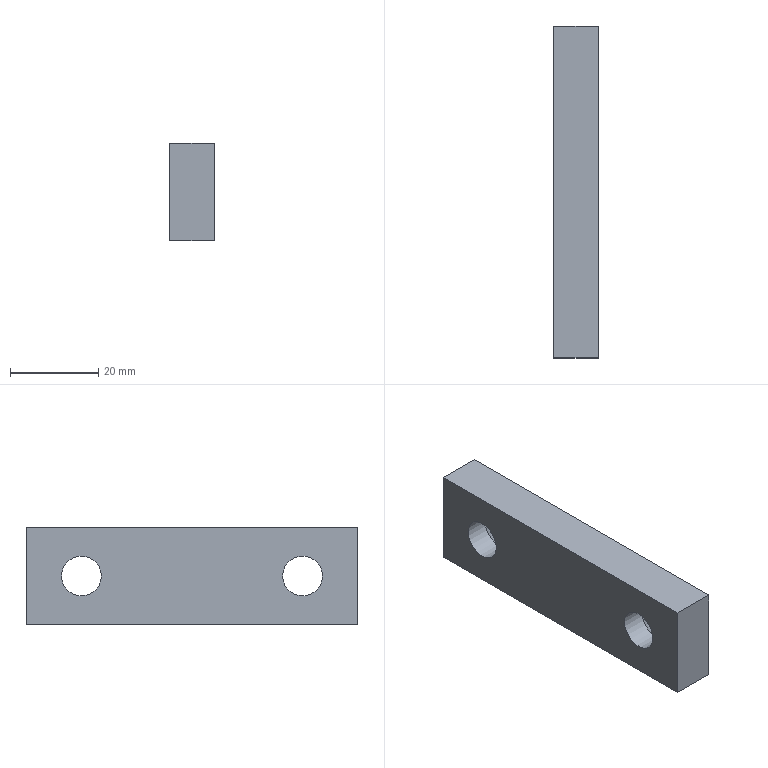Component | NX | 2_2 | 1 solid | 10 faces | box 10 x 75 x 22 mm | volume 14464 mm3 | plane 6 | cone 2 | cylinder 2 | commonest cylinder face diameters 9 x2
STEP:
#1=CARTESIAN_POINT('',(0.,0.,0.));
#2=DIRECTION('',(0.,0.,1.));
#3=DIRECTION('',(1.,0.,0.));
#4=AXIS2_PLACEMENT_3D('',#1,#2,#3);
#5=CARTESIAN_POINT('',(96.,37.5,58.5));
#6=VERTEX_POINT('',#5);
#7=CARTESIAN_POINT('',(96.,37.5,36.5));
#8=VERTEX_POINT('',#7);
#9=CARTESIAN_POINT('',(96.,37.5,58.5));
#10=DIRECTION('',(0.,0.,-1.));
#11=VECTOR('',#10,1.);
#12=LINE('',#9,#11);
#13=CARTESIAN_POINT('',(86.,37.5,58.5));
#14=DIRECTION('',(0.,-1.,0.));
#15=DIRECTION('',(1.,0.,0.));
#16=AXIS2_PLACEMENT_3D('',#13,#14,#15);
#17=PLANE('',#16);
#18=CARTESIAN_POINT('',(10.,0.));
#19=DIRECTION('',(0.,-1.));
#20=VECTOR('',#19,1.);
#21=LINE('',#18,#20);
#22=(GEOMETRIC_REPRESENTATION_CONTEXT(2)PARAMETRIC_REPRESENTATION_CONTEXT()REPRESENTATION_CONTEXT('',''));
#23=DEFINITIONAL_REPRESENTATION('',(#21),#22);
#24=PCURVE('',#17,#23);
#25=CARTESIAN_POINT('',(96.,-0.,47.5));
#26=DIRECTION('',(-1.,0.,0.));
#27=DIRECTION('',(0.,-1.,0.));
#28=AXIS2_PLACEMENT_3D('',#25,#26,#27);
#29=PLANE('',#28);
#30=CARTESIAN_POINT('',(-37.5,11.));
#31=DIRECTION('',(0.,-1.));
#32=VECTOR('',#31,1.);
#33=LINE('',#30,#32);
#34=(GEOMETRIC_REPRESENTATION_CONTEXT(2)PARAMETRIC_REPRESENTATION_CONTEXT()REPRESENTATION_CONTEXT('',''));
#35=DEFINITIONAL_REPRESENTATION('',(#33),#34);
#36=PCURVE('',#29,#35);
#37=SURFACE_CURVE('',#12,(#24,#36),.PCURVE_S1.);
#38=EDGE_CURVE('',#6,#8,#37,.T.);
#39=ORIENTED_EDGE('',*,*,#38,.T.);
#40=CARTESIAN_POINT('',(86.,37.5,36.5));
#41=VERTEX_POINT('',#40);
#42=CARTESIAN_POINT('',(86.,37.5,36.5));
#43=DIRECTION('',(1.,0.,0.));
#44=VECTOR('',#43,1.);
#45=LINE('',#42,#44);
#46=CARTESIAN_POINT('',(0.,-22.));
#47=DIRECTION('',(1.,0.));
#48=VECTOR('',#47,1.);
#49=LINE('',#46,#48);
#50=(GEOMETRIC_REPRESENTATION_CONTEXT(2)PARAMETRIC_REPRESENTATION_CONTEXT()REPRESENTATION_CONTEXT('',''));
#51=DEFINITIONAL_REPRESENTATION('',(#49),#50);
#52=PCURVE('',#17,#51);
#53=CARTESIAN_POINT('',(86.,37.5,36.5));
#54=DIRECTION('',(0.,0.,1.));
#55=DIRECTION('',(-1.,0.,0.));
#56=AXIS2_PLACEMENT_3D('',#53,#54,#55);
#57=PLANE('',#56);
#58=CARTESIAN_POINT('',(0.,0.));
#59=DIRECTION('',(-1.,0.));
#60=VECTOR('',#59,1.);
#61=LINE('',#58,#60);
#62=(GEOMETRIC_REPRESENTATION_CONTEXT(2)PARAMETRIC_REPRESENTATION_CONTEXT()REPRESENTATION_CONTEXT('',''));
#63=DEFINITIONAL_REPRESENTATION('',(#61),#62);
#64=PCURVE('',#57,#63);
#65=SURFACE_CURVE('',#45,(#52,#64),.PCURVE_S1.);
#66=EDGE_CURVE('',#41,#8,#65,.T.);
#67=ORIENTED_EDGE('',*,*,#66,.F.);
#68=CARTESIAN_POINT('',(86.,37.5,58.5));
#69=VERTEX_POINT('',#68);
#70=CARTESIAN_POINT('',(86.,37.5,58.5));
#71=DIRECTION('',(0.,0.,-1.));
#72=VECTOR('',#71,1.);
#73=LINE('',#70,#72);
#74=CARTESIAN_POINT('',(0.,0.));
#75=DIRECTION('',(0.,-1.));
#76=VECTOR('',#75,1.);
#77=LINE('',#74,#76);
#78=(GEOMETRIC_REPRESENTATION_CONTEXT(2)PARAMETRIC_REPRESENTATION_CONTEXT()REPRESENTATION_CONTEXT('',''));
#79=DEFINITIONAL_REPRESENTATION('',(#77),#78);
#80=PCURVE('',#17,#79);
#81=CARTESIAN_POINT('',(86.,-0.,47.5));
#82=DIRECTION('',(-1.,0.,0.));
#83=DIRECTION('',(0.,-1.,0.));
#84=AXIS2_PLACEMENT_3D('',#81,#82,#83);
#85=PLANE('',#84);
#86=CARTESIAN_POINT('',(-37.5,11.));
#87=DIRECTION('',(0.,-1.));
#88=VECTOR('',#87,1.);
#89=LINE('',#86,#88);
#90=(GEOMETRIC_REPRESENTATION_CONTEXT(2)PARAMETRIC_REPRESENTATION_CONTEXT()REPRESENTATION_CONTEXT('',''));
#91=DEFINITIONAL_REPRESENTATION('',(#89),#90);
#92=PCURVE('',#85,#91);
#93=SURFACE_CURVE('',#73,(#80,#92),.PCURVE_S1.);
#94=EDGE_CURVE('',#69,#41,#93,.T.);
#95=ORIENTED_EDGE('',*,*,#94,.F.);
#96=CARTESIAN_POINT('',(86.,37.5,58.5));
#97=DIRECTION('',(1.,0.,0.));
#98=VECTOR('',#97,1.);
#99=LINE('',#96,#98);
#100=CARTESIAN_POINT('',(0.,0.));
#101=DIRECTION('',(1.,0.));
#102=VECTOR('',#101,1.);
#103=LINE('',#100,#102);
#104=(GEOMETRIC_REPRESENTATION_CONTEXT(2)PARAMETRIC_REPRESENTATION_CONTEXT()REPRESENTATION_CONTEXT('',''));
#105=DEFINITIONAL_REPRESENTATION('',(#103),#104);
#106=PCURVE('',#17,#105);
#107=CARTESIAN_POINT('',(86.,-37.5,58.5));
#108=DIRECTION('',(0.,0.,-1.));
#109=DIRECTION('',(1.,0.,0.));
#110=AXIS2_PLACEMENT_3D('',#107,#108,#109);
#111=PLANE('',#110);
#112=CARTESIAN_POINT('',(0.,-75.));
#113=DIRECTION('',(1.,0.));
#114=VECTOR('',#113,1.);
#115=LINE('',#112,#114);
#116=(GEOMETRIC_REPRESENTATION_CONTEXT(2)PARAMETRIC_REPRESENTATION_CONTEXT()REPRESENTATION_CONTEXT('',''));
#117=DEFINITIONAL_REPRESENTATION('',(#115),#116);
#118=PCURVE('',#111,#117);
#119=SURFACE_CURVE('',#99,(#106,#118),.PCURVE_S1.);
#120=EDGE_CURVE('',#69,#6,#119,.T.);
#121=ORIENTED_EDGE('',*,*,#120,.T.);
#122=EDGE_LOOP('',(#39,#67,#95,#121));
#123=FACE_BOUND('',#122,.T.);
#124=ADVANCED_FACE('',(#123),#17,.F.);
#125=CARTESIAN_POINT('',(96.,-37.5,36.5));
#126=VERTEX_POINT('',#125);
#127=CARTESIAN_POINT('',(96.,37.5,36.5));
#128=DIRECTION('',(0.,-1.,0.));
#129=VECTOR('',#128,1.);
#130=LINE('',#127,#129);
#131=CARTESIAN_POINT('',(-10.,0.));
#132=DIRECTION('',(0.,1.));
#133=VECTOR('',#132,1.);
#134=LINE('',#131,#133);
#135=(GEOMETRIC_REPRESENTATION_CONTEXT(2)PARAMETRIC_REPRESENTATION_CONTEXT()REPRESENTATION_CONTEXT('',''));
#136=DEFINITIONAL_REPRESENTATION('',(#134),#135);
#137=PCURVE('',#57,#136);
#138=CARTESIAN_POINT('',(-37.5,-11.));
#139=DIRECTION('',(1.,0.));
#140=VECTOR('',#139,1.);
#141=LINE('',#138,#140);
#142=(GEOMETRIC_REPRESENTATION_CONTEXT(2)PARAMETRIC_REPRESENTATION_CONTEXT()REPRESENTATION_CONTEXT('',''));
#143=DEFINITIONAL_REPRESENTATION('',(#141),#142);
#144=PCURVE('',#29,#143);
#145=SURFACE_CURVE('',#130,(#137,#144),.PCURVE_S1.);
#146=EDGE_CURVE('',#8,#126,#145,.T.);
#147=ORIENTED_EDGE('',*,*,#146,.T.);
#148=CARTESIAN_POINT('',(86.,-37.5,36.5));
#149=VERTEX_POINT('',#148);
#150=CARTESIAN_POINT('',(86.,-37.5,36.5));
#151=DIRECTION('',(1.,0.,0.));
#152=VECTOR('',#151,1.);
#153=LINE('',#150,#152);
#154=CARTESIAN_POINT('',(0.,75.));
#155=DIRECTION('',(-1.,0.));
#156=VECTOR('',#155,1.);
#157=LINE('',#154,#156);
#158=(GEOMETRIC_REPRESENTATION_CONTEXT(2)PARAMETRIC_REPRESENTATION_CONTEXT()REPRESENTATION_CONTEXT('',''));
#159=DEFINITIONAL_REPRESENTATION('',(#157),#158);
#160=PCURVE('',#57,#159);
#161=CARTESIAN_POINT('',(86.,-37.5,36.5));
#162=DIRECTION('',(0.,1.,0.));
#163=DIRECTION('',(-1.,0.,0.));
#164=AXIS2_PLACEMENT_3D('',#161,#162,#163);
#165=PLANE('',#164);
#166=CARTESIAN_POINT('',(0.,0.));
#167=DIRECTION('',(-1.,0.));
#168=VECTOR('',#167,1.);
#169=LINE('',#166,#168);
#170=(GEOMETRIC_REPRESENTATION_CONTEXT(2)PARAMETRIC_REPRESENTATION_CONTEXT()REPRESENTATION_CONTEXT('',''));
#171=DEFINITIONAL_REPRESENTATION('',(#169),#170);
#172=PCURVE('',#165,#171);
#173=SURFACE_CURVE('',#153,(#160,#172),.PCURVE_S1.);
#174=EDGE_CURVE('',#149,#126,#173,.T.);
#175=ORIENTED_EDGE('',*,*,#174,.F.);
#176=CARTESIAN_POINT('',(86.,37.5,36.5));
#177=DIRECTION('',(0.,-1.,0.));
#178=VECTOR('',#177,1.);
#179=LINE('',#176,#178);
#180=CARTESIAN_POINT('',(0.,0.));
#181=DIRECTION('',(0.,1.));
#182=VECTOR('',#181,1.);
#183=LINE('',#180,#182);
#184=(GEOMETRIC_REPRESENTATION_CONTEXT(2)PARAMETRIC_REPRESENTATION_CONTEXT()REPRESENTATION_CONTEXT('',''));
#185=DEFINITIONAL_REPRESENTATION('',(#183),#184);
#186=PCURVE('',#57,#185);
#187=CARTESIAN_POINT('',(-37.5,-11.));
#188=DIRECTION('',(1.,0.));
#189=VECTOR('',#188,1.);
#190=LINE('',#187,#189);
#191=(GEOMETRIC_REPRESENTATION_CONTEXT(2)PARAMETRIC_REPRESENTATION_CONTEXT()REPRESENTATION_CONTEXT('',''));
#192=DEFINITIONAL_REPRESENTATION('',(#190),#191);
#193=PCURVE('',#85,#192);
#194=SURFACE_CURVE('',#179,(#186,#193),.PCURVE_S1.);
#195=EDGE_CURVE('',#41,#149,#194,.T.);
#196=ORIENTED_EDGE('',*,*,#195,.F.);
#197=ORIENTED_EDGE('',*,*,#66,.T.);
#198=EDGE_LOOP('',(#147,#175,#196,#197));
#199=FACE_BOUND('',#198,.T.);
#200=ADVANCED_FACE('',(#199),#57,.F.);
#201=CARTESIAN_POINT('',(96.,-37.5,58.5));
#202=VERTEX_POINT('',#201);
#203=CARTESIAN_POINT('',(96.,-37.5,36.5));
#204=DIRECTION('',(0.,0.,1.));
#205=VECTOR('',#204,1.);
#206=LINE('',#203,#205);
#207=CARTESIAN_POINT('',(-10.,0.));
#208=DIRECTION('',(0.,1.));
#209=VECTOR('',#208,1.);
#210=LINE('',#207,#209);
#211=(GEOMETRIC_REPRESENTATION_CONTEXT(2)PARAMETRIC_REPRESENTATION_CONTEXT()REPRESENTATION_CONTEXT('',''));
#212=DEFINITIONAL_REPRESENTATION('',(#210),#211);
#213=PCURVE('',#165,#212);
#214=CARTESIAN_POINT('',(37.5,-11.));
#215=DIRECTION('',(0.,1.));
#216=VECTOR('',#215,1.);
#217=LINE('',#214,#216);
#218=(GEOMETRIC_REPRESENTATION_CONTEXT(2)PARAMETRIC_REPRESENTATION_CONTEXT()REPRESENTATION_CONTEXT('',''));
#219=DEFINITIONAL_REPRESENTATION('',(#217),#218);
#220=PCURVE('',#29,#219);
#221=SURFACE_CURVE('',#206,(#213,#220),.PCURVE_S1.);
#222=EDGE_CURVE('',#126,#202,#221,.T.);
#223=ORIENTED_EDGE('',*,*,#222,.T.);
#224=CARTESIAN_POINT('',(86.,-37.5,58.5));
#225=VERTEX_POINT('',#224);
#226=CARTESIAN_POINT('',(86.,-37.5,58.5));
#227=DIRECTION('',(1.,0.,0.));
#228=VECTOR('',#227,1.);
#229=LINE('',#226,#228);
#230=CARTESIAN_POINT('',(0.,22.));
#231=DIRECTION('',(-1.,0.));
#232=VECTOR('',#231,1.);
#233=LINE('',#230,#232);
#234=(GEOMETRIC_REPRESENTATION_CONTEXT(2)PARAMETRIC_REPRESENTATION_CONTEXT()REPRESENTATION_CONTEXT('',''));
#235=DEFINITIONAL_REPRESENTATION('',(#233),#234);
#236=PCURVE('',#165,#235);
#237=CARTESIAN_POINT('',(0.,0.));
#238=DIRECTION('',(1.,0.));
#239=VECTOR('',#238,1.);
#240=LINE('',#237,#239);
#241=(GEOMETRIC_REPRESENTATION_CONTEXT(2)PARAMETRIC_REPRESENTATION_CONTEXT()REPRESENTATION_CONTEXT('',''));
#242=DEFINITIONAL_REPRESENTATION('',(#240),#241);
#243=PCURVE('',#111,#242);
#244=SURFACE_CURVE('',#229,(#236,#243),.PCURVE_S1.);
#245=EDGE_CURVE('',#225,#202,#244,.T.);
#246=ORIENTED_EDGE('',*,*,#245,.F.);
#247=CARTESIAN_POINT('',(86.,-37.5,36.5));
#248=DIRECTION('',(0.,0.,1.));
#249=VECTOR('',#248,1.);
#250=LINE('',#247,#249);
#251=CARTESIAN_POINT('',(0.,0.));
#252=DIRECTION('',(0.,1.));
#253=VECTOR('',#252,1.);
#254=LINE('',#251,#253);
#255=(GEOMETRIC_REPRESENTATION_CONTEXT(2)PARAMETRIC_REPRESENTATION_CONTEXT()REPRESENTATION_CONTEXT('',''));
#256=DEFINITIONAL_REPRESENTATION('',(#254),#255);
#257=PCURVE('',#165,#256);
#258=CARTESIAN_POINT('',(37.5,-11.));
#259=DIRECTION('',(0.,1.));
#260=VECTOR('',#259,1.);
#261=LINE('',#258,#260);
#262=(GEOMETRIC_REPRESENTATION_CONTEXT(2)PARAMETRIC_REPRESENTATION_CONTEXT()REPRESENTATION_CONTEXT('',''));
#263=DEFINITIONAL_REPRESENTATION('',(#261),#262);
#264=PCURVE('',#85,#263);
#265=SURFACE_CURVE('',#250,(#257,#264),.PCURVE_S1.);
#266=EDGE_CURVE('',#149,#225,#265,.T.);
#267=ORIENTED_EDGE('',*,*,#266,.F.);
#268=ORIENTED_EDGE('',*,*,#174,.T.);
#269=EDGE_LOOP('',(#223,#246,#267,#268));
#270=FACE_BOUND('',#269,.T.);
#271=ADVANCED_FACE('',(#270),#165,.F.);
#272=CARTESIAN_POINT('',(96.,-37.5,58.5));
#273=DIRECTION('',(0.,1.,0.));
#274=VECTOR('',#273,1.);
#275=LINE('',#272,#274);
#276=CARTESIAN_POINT('',(10.,0.));
#277=DIRECTION('',(0.,-1.));
#278=VECTOR('',#277,1.);
#279=LINE('',#276,#278);
#280=(GEOMETRIC_REPRESENTATION_CONTEXT(2)PARAMETRIC_REPRESENTATION_CONTEXT()REPRESENTATION_CONTEXT('',''));
#281=DEFINITIONAL_REPRESENTATION('',(#279),#280);
#282=PCURVE('',#111,#281);
#283=CARTESIAN_POINT('',(37.5,11.));
#284=DIRECTION('',(-1.,0.));
#285=VECTOR('',#284,1.);
#286=LINE('',#283,#285);
#287=(GEOMETRIC_REPRESENTATION_CONTEXT(2)PARAMETRIC_REPRESENTATION_CONTEXT()REPRESENTATION_CONTEXT('',''));
#288=DEFINITIONAL_REPRESENTATION('',(#286),#287);
#289=PCURVE('',#29,#288);
#290=SURFACE_CURVE('',#275,(#282,#289),.PCURVE_S1.);
#291=EDGE_CURVE('',#202,#6,#290,.T.);
#292=ORIENTED_EDGE('',*,*,#291,.T.);
#293=ORIENTED_EDGE('',*,*,#120,.F.);
#294=CARTESIAN_POINT('',(86.,-37.5,58.5));
#295=DIRECTION('',(0.,1.,0.));
#296=VECTOR('',#295,1.);
#297=LINE('',#294,#296);
#298=CARTESIAN_POINT('',(0.,0.));
#299=DIRECTION('',(0.,-1.));
#300=VECTOR('',#299,1.);
#301=LINE('',#298,#300);
#302=(GEOMETRIC_REPRESENTATION_CONTEXT(2)PARAMETRIC_REPRESENTATION_CONTEXT()REPRESENTATION_CONTEXT('',''));
#303=DEFINITIONAL_REPRESENTATION('',(#301),#302);
#304=PCURVE('',#111,#303);
#305=CARTESIAN_POINT('',(37.5,11.));
#306=DIRECTION('',(-1.,0.));
#307=VECTOR('',#306,1.);
#308=LINE('',#305,#307);
#309=(GEOMETRIC_REPRESENTATION_CONTEXT(2)PARAMETRIC_REPRESENTATION_CONTEXT()REPRESENTATION_CONTEXT('',''));
#310=DEFINITIONAL_REPRESENTATION('',(#308),#309);
#311=PCURVE('',#85,#310);
#312=SURFACE_CURVE('',#297,(#304,#311),.PCURVE_S1.);
#313=EDGE_CURVE('',#225,#69,#312,.T.);
#314=ORIENTED_EDGE('',*,*,#313,.F.);
#315=ORIENTED_EDGE('',*,*,#245,.T.);
#316=EDGE_LOOP('',(#292,#293,#314,#315));
#317=FACE_BOUND('',#316,.T.);
#318=ADVANCED_FACE('',(#317),#111,.F.);
#319=CARTESIAN_POINT('',(86.,-20.5,47.5));
#320=VERTEX_POINT('',#319);
#321=CARTESIAN_POINT('',(86.,-25.,47.5));
#322=DIRECTION('',(1.,0.,0.));
#323=DIRECTION('',(0.,1.,0.));
#324=AXIS2_PLACEMENT_3D('',#321,#322,#323);
#325=CIRCLE('',#324,4.5);
#326=CARTESIAN_POINT('',(20.5,0.));
#327=CARTESIAN_POINT('',(20.5,7.794));
#328=CARTESIAN_POINT('',(27.25,3.897));
#329=CARTESIAN_POINT('',(34.,0.));
#330=CARTESIAN_POINT('',(27.25,-3.897));
#331=CARTESIAN_POINT('',(20.5,-7.794));
#332=CARTESIAN_POINT('',(20.5,0.));
#333=(BOUNDED_CURVE()B_SPLINE_CURVE(2,(#326,#327,#328,#329,#330,#331,#332),.UNSPECIFIED.,.T.,.F.)B_SPLINE_CURVE_WITH_KNOTS((1,2,2,2,2,1),(-2.094,0.,2.094,4.189,6.283,8.378),.UNSPECIFIED.)CURVE()GEOMETRIC_REPRESENTATION_ITEM()RATIONAL_B_SPLINE_CURVE((1.,0.5,1.,0.5,1.,0.5,1.))REPRESENTATION_ITEM(''));
#334=(GEOMETRIC_REPRESENTATION_CONTEXT(2)PARAMETRIC_REPRESENTATION_CONTEXT()REPRESENTATION_CONTEXT('',''));
#335=DEFINITIONAL_REPRESENTATION('',(#333),#334);
#336=PCURVE('',#85,#335);
#337=CARTESIAN_POINT('',(80.151,-25.,47.5));
#338=DIRECTION('',(1.,0.,0.));
#339=DIRECTION('',(0.,1.,0.));
#340=AXIS2_PLACEMENT_3D('',#337,#338,#339);
#341=CYLINDRICAL_SURFACE('',#340,4.5);
#342=CARTESIAN_POINT('',(0.,5.849));
#343=DIRECTION('',(1.,0.));
#344=VECTOR('',#343,1.);
#345=LINE('',#342,#344);
#346=(GEOMETRIC_REPRESENTATION_CONTEXT(2)PARAMETRIC_REPRESENTATION_CONTEXT()REPRESENTATION_CONTEXT('',''));
#347=DEFINITIONAL_REPRESENTATION('',(#345),#346);
#348=PCURVE('',#341,#347);
#349=SURFACE_CURVE('',#325,(#336,#348),.PCURVE_S1.);
#350=EDGE_CURVE('',#320,#320,#349,.T.);
#351=ORIENTED_EDGE('',*,*,#350,.T.);
#352=EDGE_LOOP('',(#351));
#353=FACE_BOUND('',#352,.T.);
#354=CARTESIAN_POINT('',(86.,29.5,47.5));
#355=VERTEX_POINT('',#354);
#356=CARTESIAN_POINT('',(86.,25.,47.5));
#357=DIRECTION('',(1.,0.,0.));
#358=DIRECTION('',(0.,1.,0.));
#359=AXIS2_PLACEMENT_3D('',#356,#357,#358);
#360=CIRCLE('',#359,4.5);
#361=CARTESIAN_POINT('',(-29.5,0.));
#362=CARTESIAN_POINT('',(-29.5,7.794));
#363=CARTESIAN_POINT('',(-22.75,3.897));
#364=CARTESIAN_POINT('',(-16.,0.));
#365=CARTESIAN_POINT('',(-22.75,-3.897));
#366=CARTESIAN_POINT('',(-29.5,-7.794));
#367=CARTESIAN_POINT('',(-29.5,0.));
#368=(BOUNDED_CURVE()B_SPLINE_CURVE(2,(#361,#362,#363,#364,#365,#366,#367),.UNSPECIFIED.,.T.,.F.)B_SPLINE_CURVE_WITH_KNOTS((1,2,2,2,2,1),(-2.094,0.,2.094,4.189,6.283,8.378),.UNSPECIFIED.)CURVE()GEOMETRIC_REPRESENTATION_ITEM()RATIONAL_B_SPLINE_CURVE((1.,0.5,1.,0.5,1.,0.5,1.))REPRESENTATION_ITEM(''));
#369=(GEOMETRIC_REPRESENTATION_CONTEXT(2)PARAMETRIC_REPRESENTATION_CONTEXT()REPRESENTATION_CONTEXT('',''));
#370=DEFINITIONAL_REPRESENTATION('',(#368),#369);
#371=PCURVE('',#85,#370);
#372=CARTESIAN_POINT('',(80.151,25.,47.5));
#373=DIRECTION('',(1.,0.,0.));
#374=DIRECTION('',(0.,1.,0.));
#375=AXIS2_PLACEMENT_3D('',#372,#373,#374);
#376=CYLINDRICAL_SURFACE('',#375,4.5);
#377=CARTESIAN_POINT('',(0.,5.849));
#378=DIRECTION('',(1.,0.));
#379=VECTOR('',#378,1.);
#380=LINE('',#377,#379);
#381=(GEOMETRIC_REPRESENTATION_CONTEXT(2)PARAMETRIC_REPRESENTATION_CONTEXT()REPRESENTATION_CONTEXT('',''));
#382=DEFINITIONAL_REPRESENTATION('',(#380),#381);
#383=PCURVE('',#376,#382);
#384=SURFACE_CURVE('',#360,(#371,#383),.PCURVE_S1.);
#385=EDGE_CURVE('',#355,#355,#384,.T.);
#386=ORIENTED_EDGE('',*,*,#385,.T.);
#387=EDGE_LOOP('',(#386));
#388=FACE_BOUND('',#387,.T.);
#389=ORIENTED_EDGE('',*,*,#94,.T.);
#390=ORIENTED_EDGE('',*,*,#195,.T.);
#391=ORIENTED_EDGE('',*,*,#266,.T.);
#392=ORIENTED_EDGE('',*,*,#313,.T.);
#393=EDGE_LOOP('',(#389,#390,#391,#392));
#394=FACE_BOUND('',#393,.T.);
#395=ADVANCED_FACE('',(#353,#388,#394),#85,.T.);
#396=CARTESIAN_POINT('',(96.,-16.,47.5));
#397=VERTEX_POINT('',#396);
#398=CARTESIAN_POINT('',(96.,-25.,47.5));
#399=DIRECTION('',(1.,0.,0.));
#400=DIRECTION('',(0.,1.,0.));
#401=AXIS2_PLACEMENT_3D('',#398,#399,#400);
#402=CIRCLE('',#401,9.);
#403=CARTESIAN_POINT('',(16.,0.));
#404=CARTESIAN_POINT('',(16.,15.588));
#405=CARTESIAN_POINT('',(29.5,7.794));
#406=CARTESIAN_POINT('',(43.,0.));
#407=CARTESIAN_POINT('',(29.5,-7.794));
#408=CARTESIAN_POINT('',(16.,-15.588));
#409=CARTESIAN_POINT('',(16.,0.));
#410=(BOUNDED_CURVE()B_SPLINE_CURVE(2,(#403,#404,#405,#406,#407,#408,#409),.UNSPECIFIED.,.T.,.F.)B_SPLINE_CURVE_WITH_KNOTS((1,2,2,2,2,1),(-2.094,0.,2.094,4.189,6.283,8.378),.UNSPECIFIED.)CURVE()GEOMETRIC_REPRESENTATION_ITEM()RATIONAL_B_SPLINE_CURVE((1.,0.5,1.,0.5,1.,0.5,1.))REPRESENTATION_ITEM(''));
#411=(GEOMETRIC_REPRESENTATION_CONTEXT(2)PARAMETRIC_REPRESENTATION_CONTEXT()REPRESENTATION_CONTEXT('',''));
#412=DEFINITIONAL_REPRESENTATION('',(#410),#411);
#413=PCURVE('',#29,#412);
#414=CARTESIAN_POINT('',(96.,-25.,47.5));
#415=DIRECTION('',(1.,0.,0.));
#416=DIRECTION('',(0.,1.,0.));
#417=AXIS2_PLACEMENT_3D('',#414,#415,#416);
#418=CONICAL_SURFACE('',#417,9.,0.7854);
#419=CARTESIAN_POINT('',(0.,0.));
#420=DIRECTION('',(1.,0.));
#421=VECTOR('',#420,1.);
#422=LINE('',#419,#421);
#423=(GEOMETRIC_REPRESENTATION_CONTEXT(2)PARAMETRIC_REPRESENTATION_CONTEXT()REPRESENTATION_CONTEXT('',''));
#424=DEFINITIONAL_REPRESENTATION('',(#422),#423);
#425=PCURVE('',#418,#424);
#426=SURFACE_CURVE('',#402,(#413,#425),.PCURVE_S1.);
#427=EDGE_CURVE('',#397,#397,#426,.T.);
#428=ORIENTED_EDGE('',*,*,#427,.F.);
#429=EDGE_LOOP('',(#428));
#430=FACE_BOUND('',#429,.T.);
#431=CARTESIAN_POINT('',(96.,34.,47.5));
#432=VERTEX_POINT('',#431);
#433=CARTESIAN_POINT('',(96.,25.,47.5));
#434=DIRECTION('',(1.,0.,0.));
#435=DIRECTION('',(0.,1.,0.));
#436=AXIS2_PLACEMENT_3D('',#433,#434,#435);
#437=CIRCLE('',#436,9.);
#438=CARTESIAN_POINT('',(-34.,0.));
#439=CARTESIAN_POINT('',(-34.,15.588));
#440=CARTESIAN_POINT('',(-20.5,7.794));
#441=CARTESIAN_POINT('',(-7.,0.));
#442=CARTESIAN_POINT('',(-20.5,-7.794));
#443=CARTESIAN_POINT('',(-34.,-15.588));
#444=CARTESIAN_POINT('',(-34.,0.));
#445=(BOUNDED_CURVE()B_SPLINE_CURVE(2,(#438,#439,#440,#441,#442,#443,#444),.UNSPECIFIED.,.T.,.F.)B_SPLINE_CURVE_WITH_KNOTS((1,2,2,2,2,1),(-2.094,0.,2.094,4.189,6.283,8.378),.UNSPECIFIED.)CURVE()GEOMETRIC_REPRESENTATION_ITEM()RATIONAL_B_SPLINE_CURVE((1.,0.5,1.,0.5,1.,0.5,1.))REPRESENTATION_ITEM(''));
#446=(GEOMETRIC_REPRESENTATION_CONTEXT(2)PARAMETRIC_REPRESENTATION_CONTEXT()REPRESENTATION_CONTEXT('',''));
#447=DEFINITIONAL_REPRESENTATION('',(#445),#446);
#448=PCURVE('',#29,#447);
#449=CARTESIAN_POINT('',(96.,25.,47.5));
#450=DIRECTION('',(1.,0.,0.));
#451=DIRECTION('',(0.,1.,0.));
#452=AXIS2_PLACEMENT_3D('',#449,#450,#451);
#453=CONICAL_SURFACE('',#452,9.,0.7854);
#454=CARTESIAN_POINT('',(0.,0.));
#455=DIRECTION('',(1.,0.));
#456=VECTOR('',#455,1.);
#457=LINE('',#454,#456);
#458=(GEOMETRIC_REPRESENTATION_CONTEXT(2)PARAMETRIC_REPRESENTATION_CONTEXT()REPRESENTATION_CONTEXT('',''));
#459=DEFINITIONAL_REPRESENTATION('',(#457),#458);
#460=PCURVE('',#453,#459);
#461=SURFACE_CURVE('',#437,(#448,#460),.PCURVE_S1.);
#462=EDGE_CURVE('',#432,#432,#461,.T.);
#463=ORIENTED_EDGE('',*,*,#462,.F.);
#464=EDGE_LOOP('',(#463));
#465=FACE_BOUND('',#464,.T.);
#466=ORIENTED_EDGE('',*,*,#38,.F.);
#467=ORIENTED_EDGE('',*,*,#291,.F.);
#468=ORIENTED_EDGE('',*,*,#222,.F.);
#469=ORIENTED_EDGE('',*,*,#146,.F.);
#470=EDGE_LOOP('',(#466,#467,#468,#469));
#471=FACE_BOUND('',#470,.T.);
#472=ADVANCED_FACE('',(#430,#465,#471),#29,.F.);
#473=CARTESIAN_POINT('',(91.5,29.5,47.5));
#474=VERTEX_POINT('',#473);
#475=CARTESIAN_POINT('',(91.5,25.,47.5));
#476=DIRECTION('',(-1.,0.,0.));
#477=DIRECTION('',(0.,1.,0.));
#478=AXIS2_PLACEMENT_3D('',#475,#476,#477);
#479=CIRCLE('',#478,4.5);
#480=CARTESIAN_POINT('',(6.283,-4.5));
#481=DIRECTION('',(-1.,0.));
#482=VECTOR('',#481,1.);
#483=LINE('',#480,#482);
#484=(GEOMETRIC_REPRESENTATION_CONTEXT(2)PARAMETRIC_REPRESENTATION_CONTEXT()REPRESENTATION_CONTEXT('',''));
#485=DEFINITIONAL_REPRESENTATION('',(#483),#484);
#486=PCURVE('',#453,#485);
#487=CARTESIAN_POINT('',(6.283,11.349));
#488=DIRECTION('',(-1.,0.));
#489=VECTOR('',#488,1.);
#490=LINE('',#487,#489);
#491=(GEOMETRIC_REPRESENTATION_CONTEXT(2)PARAMETRIC_REPRESENTATION_CONTEXT()REPRESENTATION_CONTEXT('',''));
#492=DEFINITIONAL_REPRESENTATION('',(#490),#491);
#493=PCURVE('',#376,#492);
#494=SURFACE_CURVE('',#479,(#486,#493),.PCURVE_S1.);
#495=EDGE_CURVE('',#474,#474,#494,.T.);
#496=ORIENTED_EDGE('',*,*,#495,.F.);
#497=CARTESIAN_POINT('',(91.5,29.5,47.5));
#498=CARTESIAN_POINT('',(96.,34.,47.5));
#499=B_SPLINE_CURVE_WITH_KNOTS('',1,(#497,#498),.UNSPECIFIED.,.F.,.F.,(2,2),(-6.364,0.),.PIECEWISE_BEZIER_KNOTS.);
#500=CARTESIAN_POINT('',(6.283,0.));
#501=DIRECTION('',(0.,1.));
#502=VECTOR('',#501,1.);
#503=LINE('',#500,#502);
#504=(GEOMETRIC_REPRESENTATION_CONTEXT(2)PARAMETRIC_REPRESENTATION_CONTEXT()REPRESENTATION_CONTEXT('',''));
#505=DEFINITIONAL_REPRESENTATION('',(#503),#504);
#506=PCURVE('',#453,#505);
#507=CARTESIAN_POINT('',(0.,0.));
#508=DIRECTION('',(0.,1.));
#509=VECTOR('',#508,1.);
#510=LINE('',#507,#509);
#511=(GEOMETRIC_REPRESENTATION_CONTEXT(2)PARAMETRIC_REPRESENTATION_CONTEXT()REPRESENTATION_CONTEXT('',''));
#512=DEFINITIONAL_REPRESENTATION('',(#510),#511);
#513=PCURVE('',#453,#512);
#514=SEAM_CURVE('',#499,(#506,#513),.PCURVE_S1.);
#515=EDGE_CURVE('',#474,#432,#514,.T.);
#516=ORIENTED_EDGE('',*,*,#515,.T.);
#517=ORIENTED_EDGE('',*,*,#462,.F.);
#518=ORIENTED_EDGE('',*,*,#515,.F.);
#519=EDGE_LOOP('',(#496,#516,#517,#518));
#520=FACE_BOUND('',#519,.F.);
#521=ADVANCED_FACE('',(#520),#453,.F.);
#522=ORIENTED_EDGE('',*,*,#385,.T.);
#523=CARTESIAN_POINT('',(86.,29.5,47.5));
#524=CARTESIAN_POINT('',(91.5,29.5,47.5));
#525=B_SPLINE_CURVE_WITH_KNOTS('',1,(#523,#524),.UNSPECIFIED.,.F.,.F.,(2,2),(5.849,11.349),.PIECEWISE_BEZIER_KNOTS.);
#526=CARTESIAN_POINT('',(6.283,0.));
#527=DIRECTION('',(0.,1.));
#528=VECTOR('',#527,1.);
#529=LINE('',#526,#528);
#530=(GEOMETRIC_REPRESENTATION_CONTEXT(2)PARAMETRIC_REPRESENTATION_CONTEXT()REPRESENTATION_CONTEXT('',''));
#531=DEFINITIONAL_REPRESENTATION('',(#529),#530);
#532=PCURVE('',#376,#531);
#533=CARTESIAN_POINT('',(0.,0.));
#534=DIRECTION('',(0.,1.));
#535=VECTOR('',#534,1.);
#536=LINE('',#533,#535);
#537=(GEOMETRIC_REPRESENTATION_CONTEXT(2)PARAMETRIC_REPRESENTATION_CONTEXT()REPRESENTATION_CONTEXT('',''));
#538=DEFINITIONAL_REPRESENTATION('',(#536),#537);
#539=PCURVE('',#376,#538);
#540=SEAM_CURVE('',#525,(#532,#539),.PCURVE_S1.);
#541=EDGE_CURVE('',#355,#474,#540,.T.);
#542=ORIENTED_EDGE('',*,*,#541,.T.);
#543=ORIENTED_EDGE('',*,*,#495,.T.);
#544=ORIENTED_EDGE('',*,*,#541,.F.);
#545=EDGE_LOOP('',(#522,#542,#543,#544));
#546=FACE_BOUND('',#545,.F.);
#547=ADVANCED_FACE('',(#546),#376,.F.);
#548=CARTESIAN_POINT('',(91.5,-20.5,47.5));
#549=VERTEX_POINT('',#548);
#550=CARTESIAN_POINT('',(91.5,-25.,47.5));
#551=DIRECTION('',(1.,0.,0.));
#552=DIRECTION('',(0.,1.,0.));
#553=AXIS2_PLACEMENT_3D('',#550,#551,#552);
#554=CIRCLE('',#553,4.5);
#555=CARTESIAN_POINT('',(0.,-4.5));
#556=DIRECTION('',(1.,0.));
#557=VECTOR('',#556,1.);
#558=LINE('',#555,#557);
#559=(GEOMETRIC_REPRESENTATION_CONTEXT(2)PARAMETRIC_REPRESENTATION_CONTEXT()REPRESENTATION_CONTEXT('',''));
#560=DEFINITIONAL_REPRESENTATION('',(#558),#559);
#561=PCURVE('',#418,#560);
#562=CARTESIAN_POINT('',(0.,11.349));
#563=DIRECTION('',(1.,0.));
#564=VECTOR('',#563,1.);
#565=LINE('',#562,#564);
#566=(GEOMETRIC_REPRESENTATION_CONTEXT(2)PARAMETRIC_REPRESENTATION_CONTEXT()REPRESENTATION_CONTEXT('',''));
#567=DEFINITIONAL_REPRESENTATION('',(#565),#566);
#568=PCURVE('',#341,#567);
#569=SURFACE_CURVE('',#554,(#561,#568),.PCURVE_S1.);
#570=EDGE_CURVE('',#549,#549,#569,.T.);
#571=ORIENTED_EDGE('',*,*,#570,.T.);
#572=CARTESIAN_POINT('',(91.5,-20.5,47.5));
#573=CARTESIAN_POINT('',(96.,-16.,47.5));
#574=B_SPLINE_CURVE_WITH_KNOTS('',1,(#572,#573),.UNSPECIFIED.,.F.,.F.,(2,2),(-6.364,0.),.PIECEWISE_BEZIER_KNOTS.);
#575=CARTESIAN_POINT('',(6.283,0.));
#576=DIRECTION('',(0.,1.));
#577=VECTOR('',#576,1.);
#578=LINE('',#575,#577);
#579=(GEOMETRIC_REPRESENTATION_CONTEXT(2)PARAMETRIC_REPRESENTATION_CONTEXT()REPRESENTATION_CONTEXT('',''));
#580=DEFINITIONAL_REPRESENTATION('',(#578),#579);
#581=PCURVE('',#418,#580);
#582=CARTESIAN_POINT('',(0.,0.));
#583=DIRECTION('',(0.,1.));
#584=VECTOR('',#583,1.);
#585=LINE('',#582,#584);
#586=(GEOMETRIC_REPRESENTATION_CONTEXT(2)PARAMETRIC_REPRESENTATION_CONTEXT()REPRESENTATION_CONTEXT('',''));
#587=DEFINITIONAL_REPRESENTATION('',(#585),#586);
#588=PCURVE('',#418,#587);
#589=SEAM_CURVE('',#574,(#581,#588),.PCURVE_S1.);
#590=EDGE_CURVE('',#549,#397,#589,.T.);
#591=ORIENTED_EDGE('',*,*,#590,.T.);
#592=ORIENTED_EDGE('',*,*,#427,.F.);
#593=ORIENTED_EDGE('',*,*,#590,.F.);
#594=EDGE_LOOP('',(#571,#591,#592,#593));
#595=FACE_BOUND('',#594,.F.);
#596=ADVANCED_FACE('',(#595),#418,.F.);
#597=ORIENTED_EDGE('',*,*,#350,.T.);
#598=CARTESIAN_POINT('',(86.,-20.5,47.5));
#599=CARTESIAN_POINT('',(91.5,-20.5,47.5));
#600=B_SPLINE_CURVE_WITH_KNOTS('',1,(#598,#599),.UNSPECIFIED.,.F.,.F.,(2,2),(5.849,11.349),.PIECEWISE_BEZIER_KNOTS.);
#601=CARTESIAN_POINT('',(6.283,0.));
#602=DIRECTION('',(0.,1.));
#603=VECTOR('',#602,1.);
#604=LINE('',#601,#603);
#605=(GEOMETRIC_REPRESENTATION_CONTEXT(2)PARAMETRIC_REPRESENTATION_CONTEXT()REPRESENTATION_CONTEXT('',''));
#606=DEFINITIONAL_REPRESENTATION('',(#604),#605);
#607=PCURVE('',#341,#606);
#608=CARTESIAN_POINT('',(0.,0.));
#609=DIRECTION('',(0.,1.));
#610=VECTOR('',#609,1.);
#611=LINE('',#608,#610);
#612=(GEOMETRIC_REPRESENTATION_CONTEXT(2)PARAMETRIC_REPRESENTATION_CONTEXT()REPRESENTATION_CONTEXT('',''));
#613=DEFINITIONAL_REPRESENTATION('',(#611),#612);
#614=PCURVE('',#341,#613);
#615=SEAM_CURVE('',#600,(#607,#614),.PCURVE_S1.);
#616=EDGE_CURVE('',#320,#549,#615,.T.);
#617=ORIENTED_EDGE('',*,*,#616,.T.);
#618=ORIENTED_EDGE('',*,*,#570,.F.);
#619=ORIENTED_EDGE('',*,*,#616,.F.);
#620=EDGE_LOOP('',(#597,#617,#618,#619));
#621=FACE_BOUND('',#620,.F.);
#622=ADVANCED_FACE('',(#621),#341,.F.);
#623=CLOSED_SHELL('',(#124,#200,#271,#318,#395,#472,#521,#547,#596,#622));
#624=MANIFOLD_SOLID_BREP('',#623);
#625=(LENGTH_UNIT()NAMED_UNIT(*)SI_UNIT(.MILLI.,.METRE.));
#626=UNCERTAINTY_MEASURE_WITH_UNIT(LENGTH_MEASURE(0.000005),#625,'','');
#627=(NAMED_UNIT(*)PLANE_ANGLE_UNIT()SI_UNIT($,.RADIAN.));
#628=(NAMED_UNIT(*)SI_UNIT($,.STERADIAN.)SOLID_ANGLE_UNIT());
#629=(GEOMETRIC_REPRESENTATION_CONTEXT(3)GLOBAL_UNCERTAINTY_ASSIGNED_CONTEXT((#626))GLOBAL_UNIT_ASSIGNED_CONTEXT((#625,#627,#628))REPRESENTATION_CONTEXT('',''));
#630=ADVANCED_BREP_SHAPE_REPRESENTATION('',(#4,#624),#629);